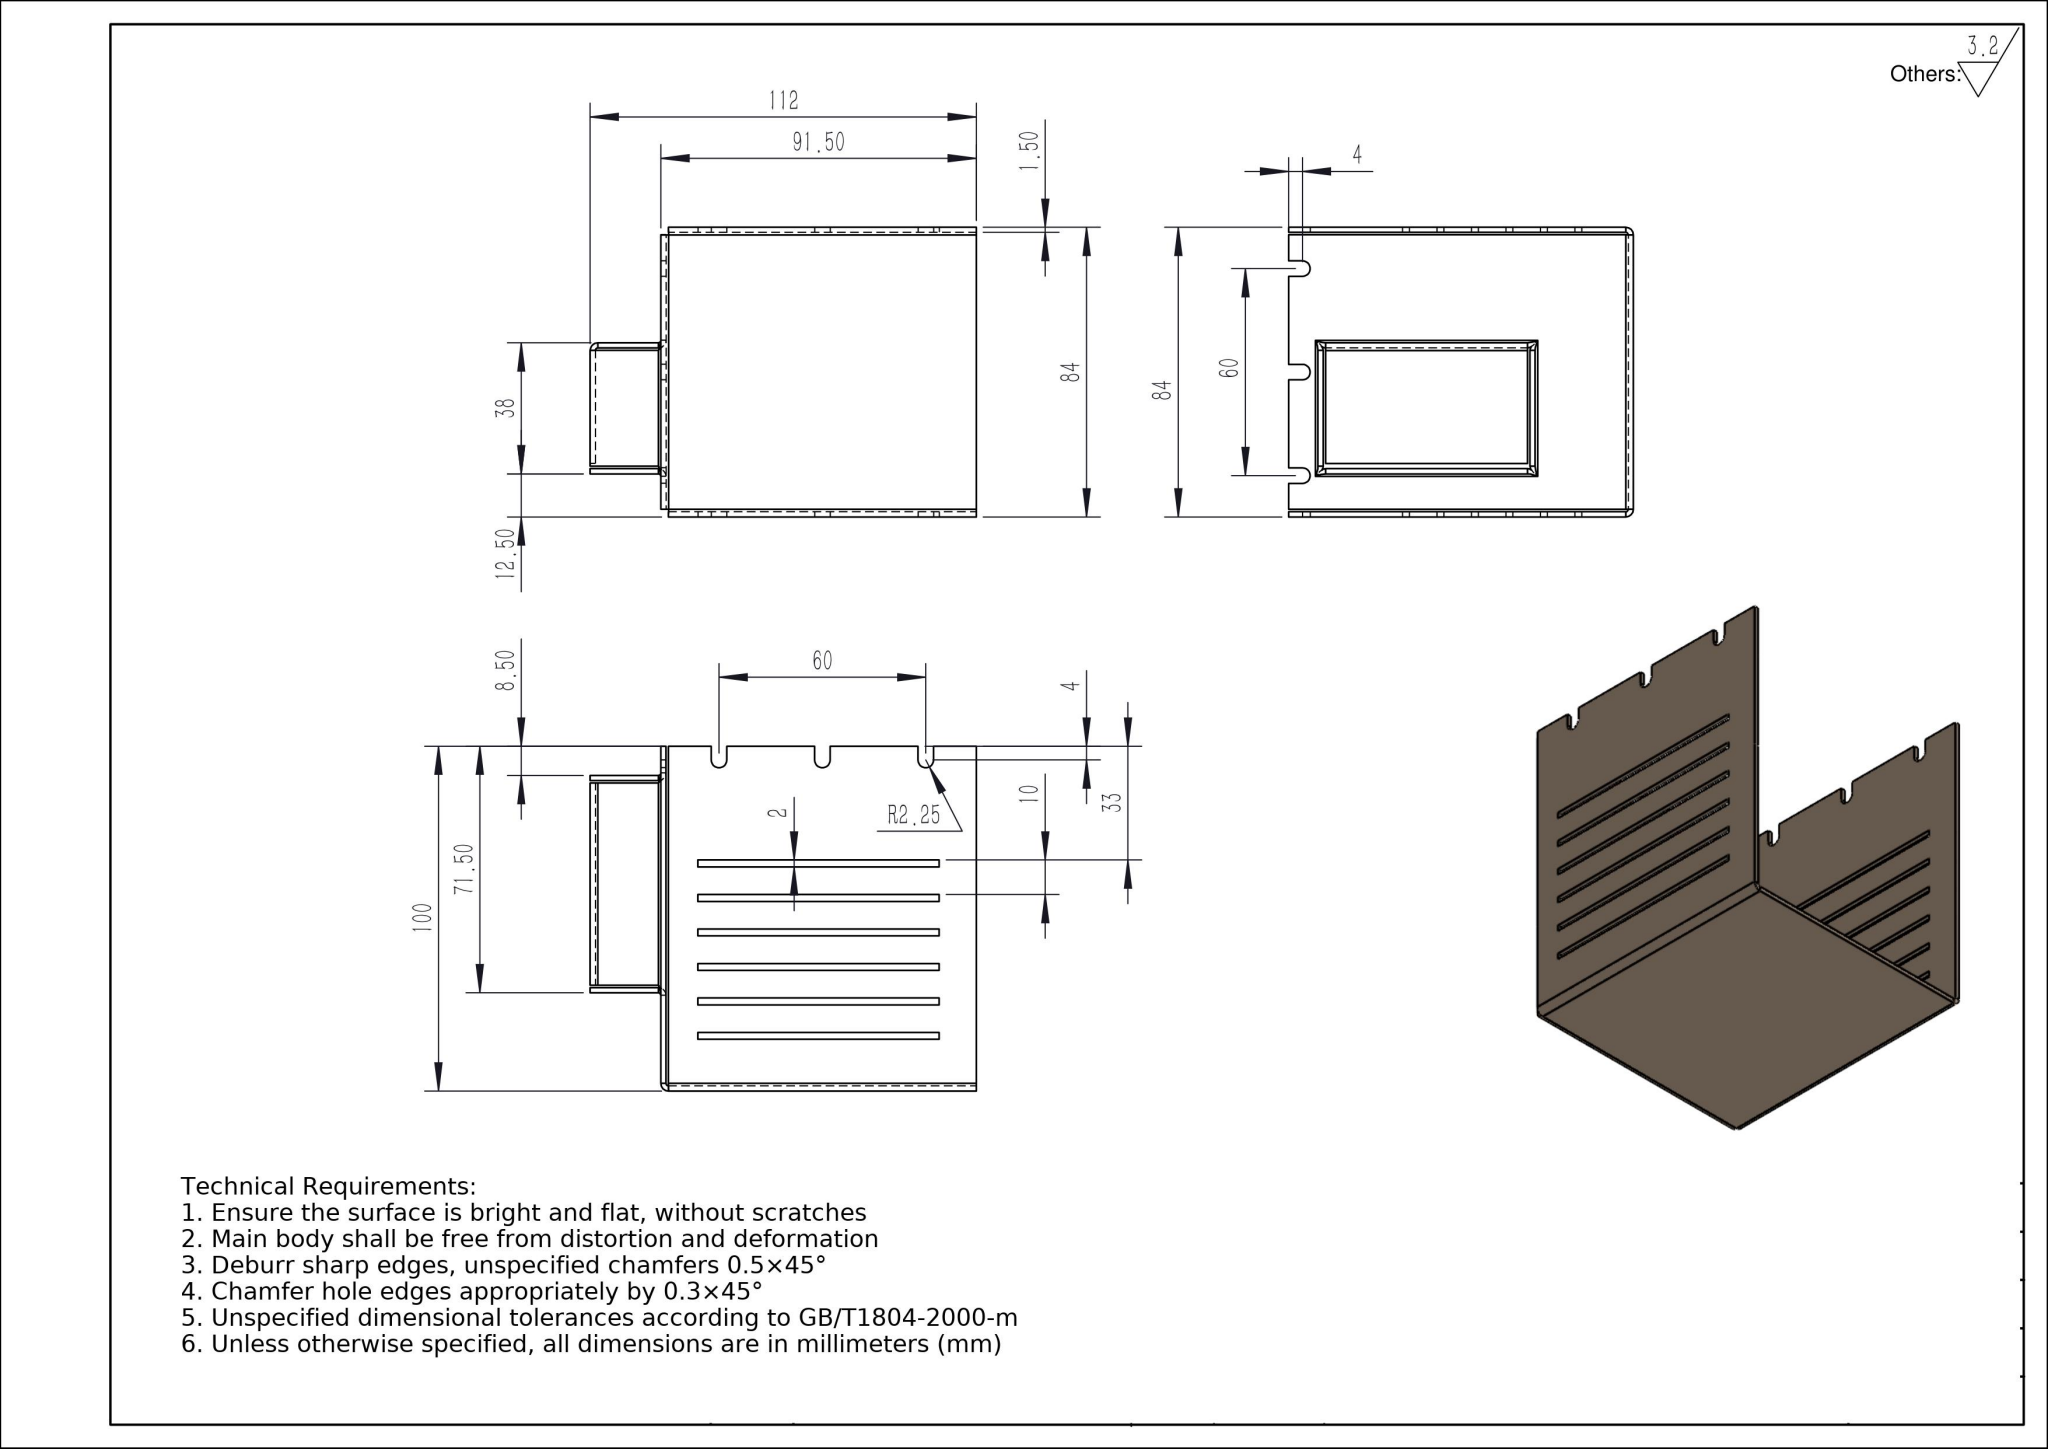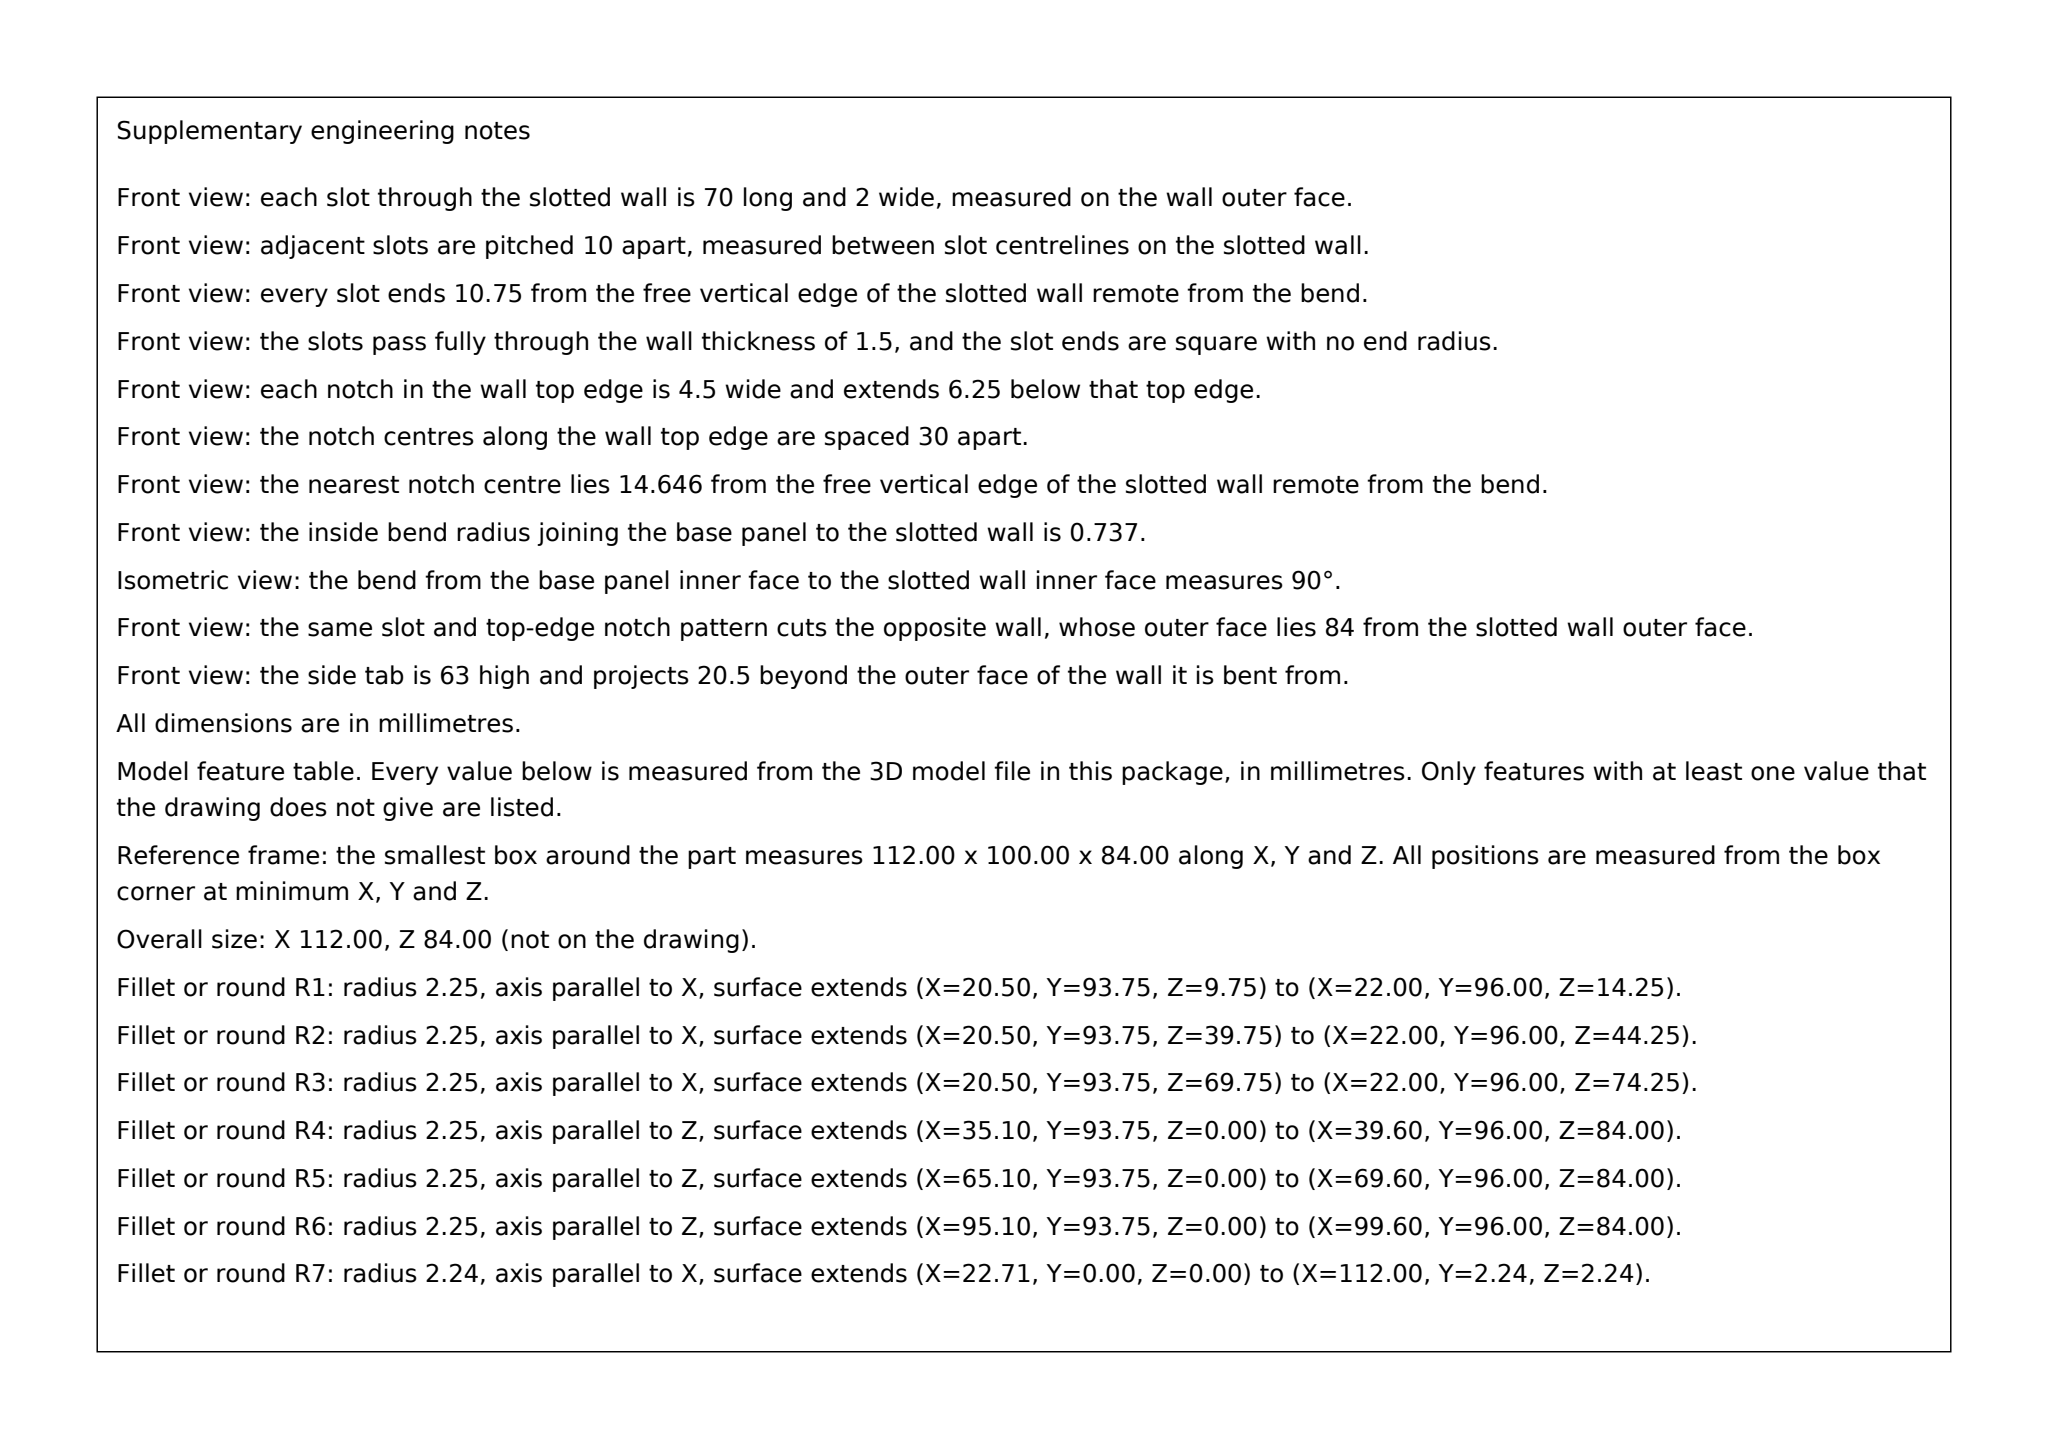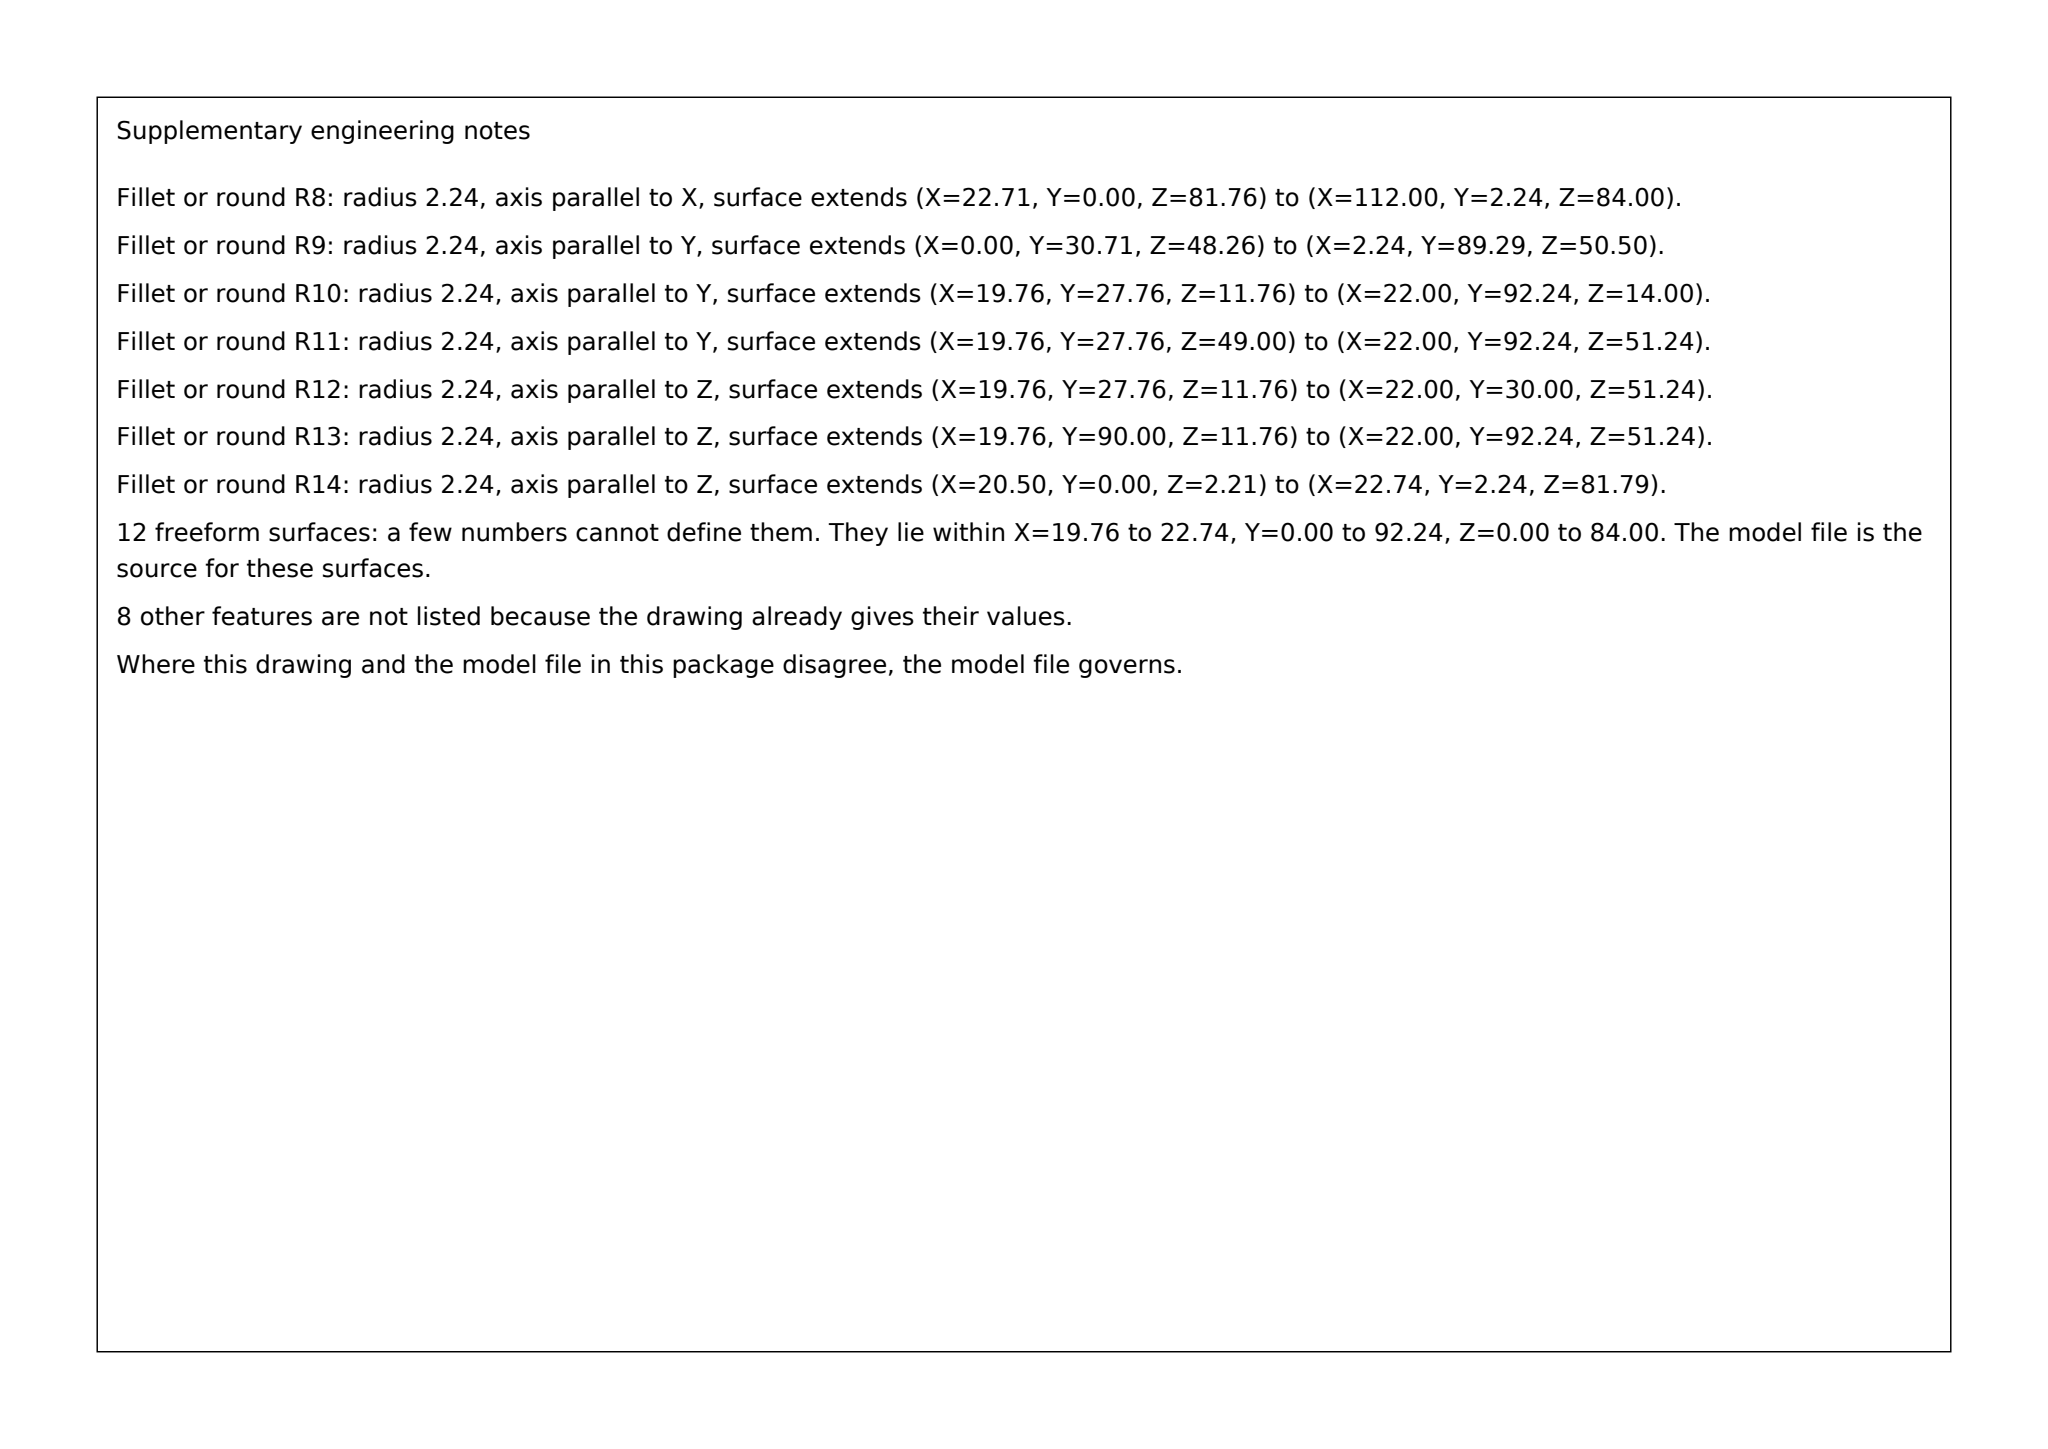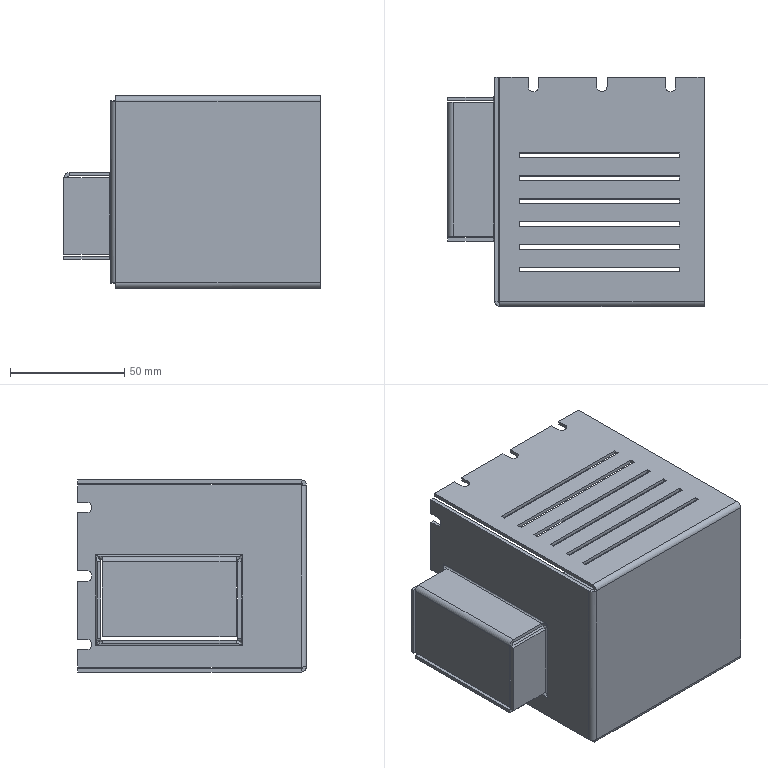Part | SolidWorks | mm | 1 solid | 161 faces | box 112 x 100 x 84 mm | volume 51764 mm3 | plane 121 | cylinder 28 | spline 12 | commonest cylinder face diameters 4.5 x12 4.473 x8 1.473 x8
Drawing notes:
SHEET THK 1.5; ALL BENDS INSIDE R0.75, OUTSIDE R2.25 | from the solid: Wall planes 1.5 apart (x 0.0/1.5, y 0.02/1.52); bend cyl Ø1.473 inner, Ø4.473 outer
LOUVER SLOT 70 LG X 2 WIDE, 10 PITCH, 6X EA PANEL, 12 TOTAL | from the solid: 12 slot faces at x=31.25 and 12 at x=101.25; y pairs 15.02/17.02...65.02/67.02 = 2 wide, 10 pitch
SIDE POCKET 63 X 38 OUTER, ID 60 X 35, 20.50 DP | from the solid: y 28.52-91.52=63 / 30.02-90.02=60; z 12.52-50.52=38 / 14.02-49.02=35; x 0-20.5 depth